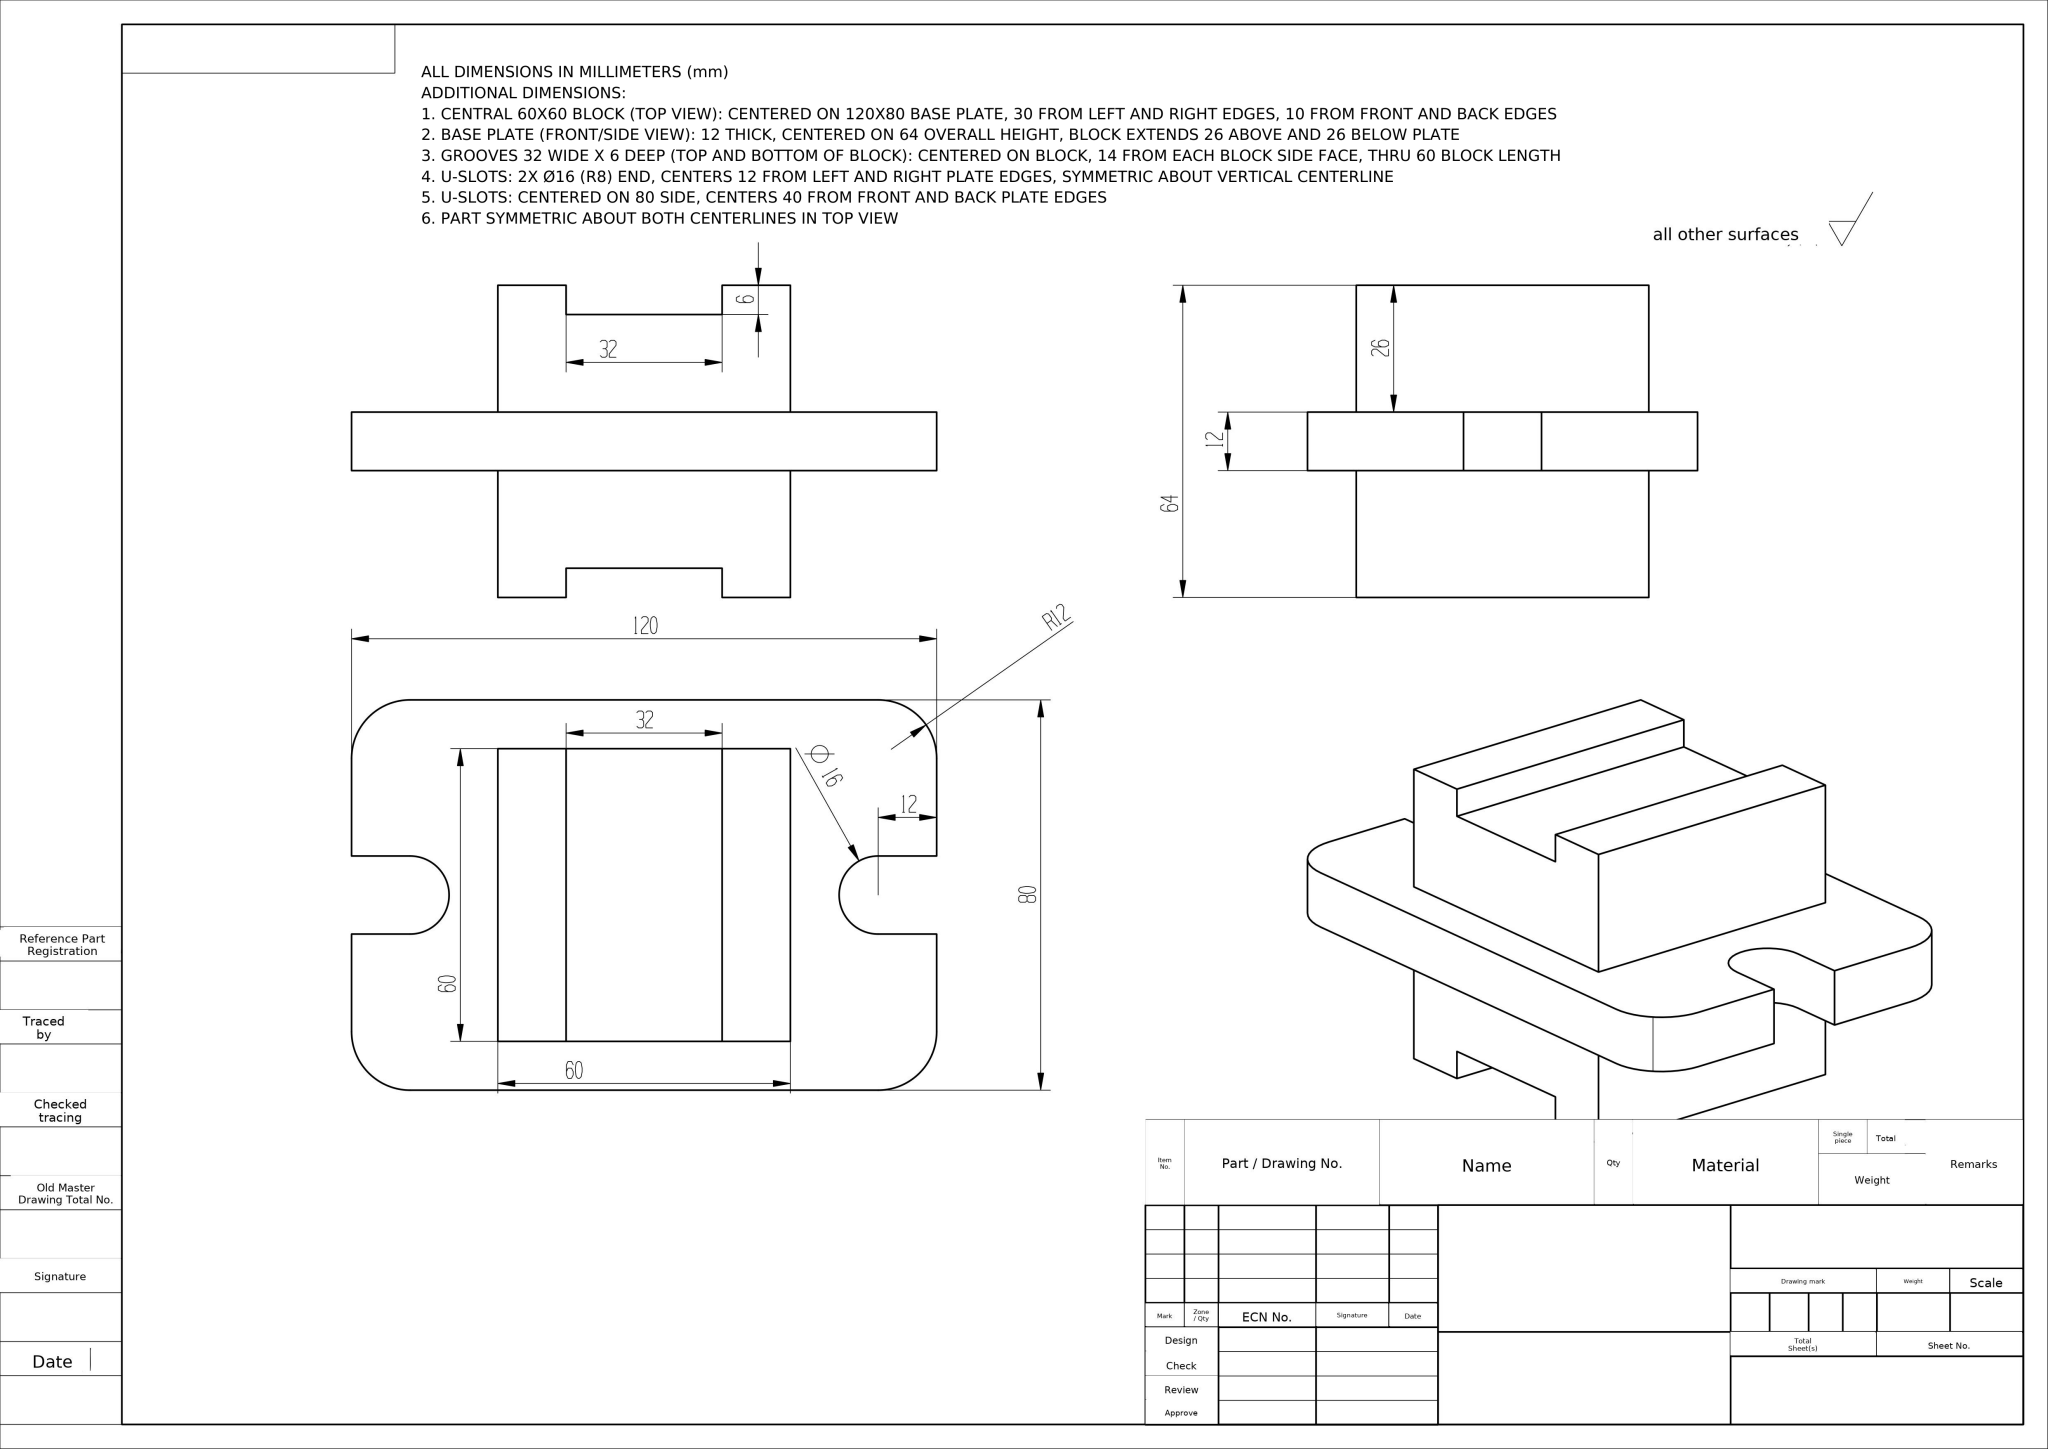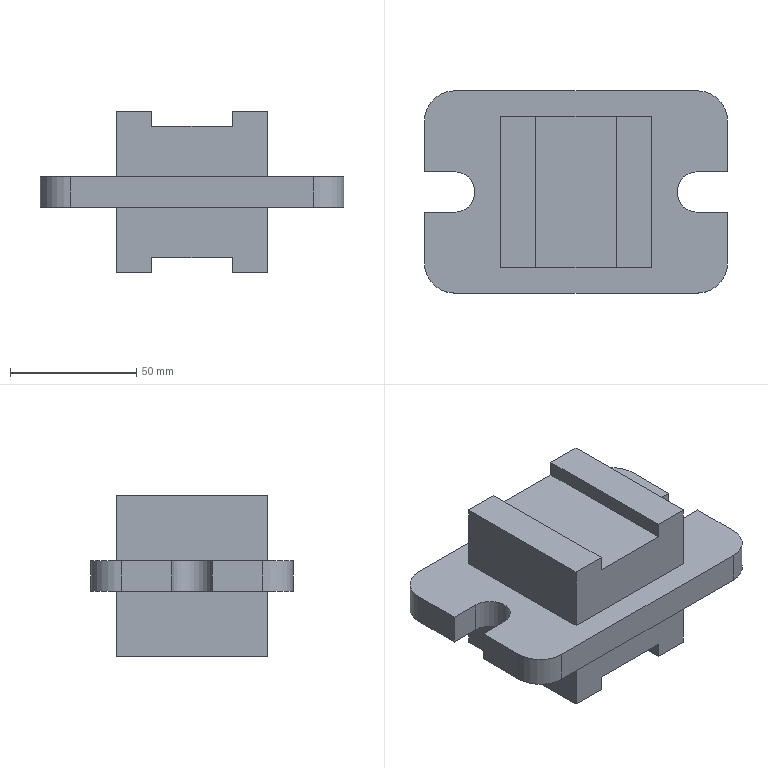Part | NX | mm | 1 solid | 36 faces | box 120 x 80 x 64 mm | volume 270856 mm3 | plane 30 | cylinder 6 | commonest cylinder face diameters 24 x4 16 x2